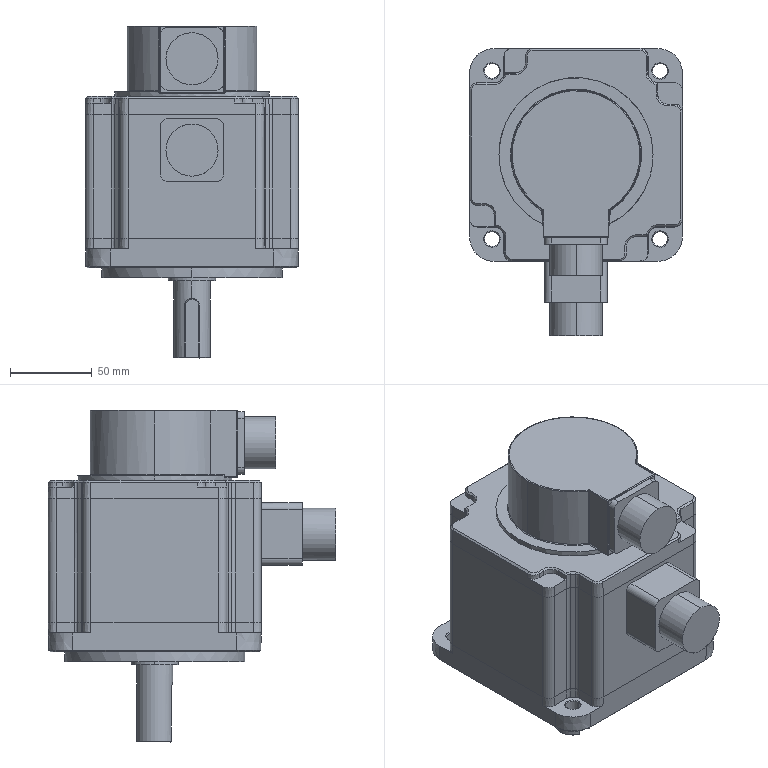Component | SolidWorks | ServoMotor(Delta)ENCODE-Rex1320fs-1 | 1 solid | 288 faces | volume 1917840 mm3 | plane 123 | cone 90 | cylinder 64 | spline 11 | commonest cylinder face diameters 1 x12 8 x9 9 x8 10 x8 6 x8 31.75 x4 29 x4 79 x3